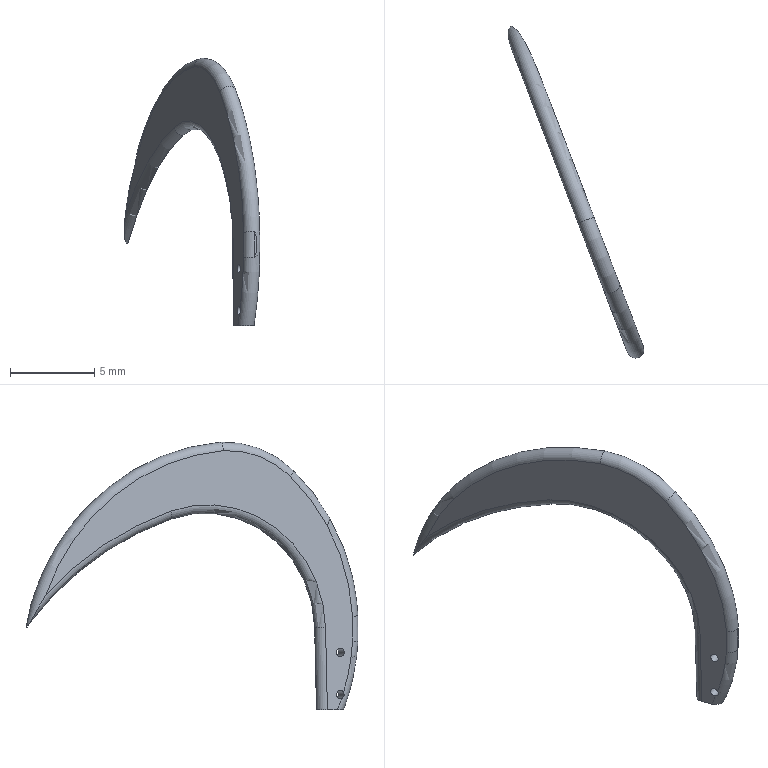Component | NX | CUTTING_BLADE | 1 solid | 16 faces | box 8.06 x 19.66 x 15.86 mm | volume 81 mm3 | torus 7 | cylinder 5 | plane 4 | commonest cylinder face diameters 1 x2 0.5 x2 12 x1
STEP:
#1=VALUE_REPRESENTATION_ITEM('',COUNT_MEASURE(0.));
#2=(LENGTH_UNIT()NAMED_UNIT(*)SI_UNIT(.MILLI.,.METRE.));
#3=UNCERTAINTY_MEASURE_WITH_UNIT(LENGTH_MEASURE(0.0508),#2,'','');
#4=(NAMED_UNIT(*)PLANE_ANGLE_UNIT()SI_UNIT($,.RADIAN.));
#5=PLANE_ANGLE_MEASURE_WITH_UNIT(PLANE_ANGLE_MEASURE(0.01745),#4);
#6=DIMENSIONAL_EXPONENTS(0.,0.,0.,0.,0.,0.,0.);
#7=(CONVERSION_BASED_UNIT('',#5)NAMED_UNIT(#6)PLANE_ANGLE_UNIT());
#8=(NAMED_UNIT(*)SI_UNIT($,.STERADIAN.)SOLID_ANGLE_UNIT());
#9=(GEOMETRIC_REPRESENTATION_CONTEXT(3)GLOBAL_UNCERTAINTY_ASSIGNED_CONTEXT((#3))GLOBAL_UNIT_ASSIGNED_CONTEXT((#2,#7,#8))REPRESENTATION_CONTEXT('',''));
#10=REPRESENTATION('',(#1),#9);
#11=VALUE_REPRESENTATION_ITEM('',COUNT_MEASURE(0.));
#12=REPRESENTATION('',(#11),#9);
#13=CARTESIAN_POINT('',(0.,0.,0.));
#14=DIRECTION('',(0.,0.,1.));
#15=DIRECTION('',(1.,0.,0.));
#16=AXIS2_PLACEMENT_3D('',#13,#14,#15);
#17=SHAPE_REPRESENTATION('',(#16),#9);
#18=CARTESIAN_POINT('',(-0.7584,2.547,-2.1));
#19=VERTEX_POINT('',#18);
#20=CARTESIAN_POINT('',(-0.8475,2.781,-2.1));
#21=DIRECTION('',(-0.9342,-0.3566,0.));
#22=DIRECTION('',(0.3566,-0.9342,0.));
#23=AXIS2_PLACEMENT_3D('',#20,#21,#22);
#24=CIRCLE('',#23,0.25);
#25=EDGE_CURVE('',#19,#19,#24,.T.);
#26=ORIENTED_EDGE('',*,*,#25,.F.);
#27=EDGE_LOOP('',(#26));
#28=FACE_BOUND('',#27,.T.);
#29=CARTESIAN_POINT('',(-1.18,3.651,-0.6366));
#30=VERTEX_POINT('',#29);
#31=CARTESIAN_POINT('',(-1.138,3.542,-5.5));
#32=VERTEX_POINT('',#31);
#33=CARTESIAN_POINT('',(-1.078,3.384,-12.534));
#34=DIRECTION('',(0.008553,-0.02241,-0.9997));
#35=VECTOR('',#34,1.);
#36=LINE('',#33,#35);
#37=EDGE_CURVE('',#30,#32,#36,.T.);
#38=ORIENTED_EDGE('',*,*,#37,.T.);
#39=CARTESIAN_POINT('',(-0.9125,2.951,-5.5));
#40=VERTEX_POINT('',#39);
#41=CARTESIAN_POINT('',(-2.44,6.953,-5.5));
#42=DIRECTION('',(0.3566,-0.9342,0.));
#43=VECTOR('',#42,1.);
#44=LINE('',#41,#43);
#45=EDGE_CURVE('',#32,#40,#44,.T.);
#46=ORIENTED_EDGE('',*,*,#45,.T.);
#47=CARTESIAN_POINT('',(-0.8194,2.707,-4.837));
#48=VERTEX_POINT('',#47);
#49=CARTESIAN_POINT('',(-4.918,13.443,-0.6896));
#50=DIRECTION('',(-0.9342,-0.3566,0.));
#51=DIRECTION('',(0.,0.,1.));
#52=AXIS2_PLACEMENT_3D('',#49,#50,#51);
#53=CIRCLE('',#52,12.217);
#54=EDGE_CURVE('',#40,#48,#53,.T.);
#55=ORIENTED_EDGE('',*,*,#54,.T.);
#56=CARTESIAN_POINT('',(-0.7734,2.587,-4.461));
#57=VERTEX_POINT('',#56);
#58=CARTESIAN_POINT('',(-0.8475,2.781,-4.6));
#59=DIRECTION('',(-0.9342,-0.3566,0.));
#60=DIRECTION('',(0.3566,-0.9342,0.));
#61=AXIS2_PLACEMENT_3D('',#58,#59,#60);
#62=CIRCLE('',#61,0.25);
#63=EDGE_CURVE('',#57,#48,#62,.T.);
#64=ORIENTED_EDGE('',*,*,#63,.F.);
#65=CARTESIAN_POINT('',(-0.5687,2.05,-1.433));
#66=VERTEX_POINT('',#65);
#67=CARTESIAN_POINT('',(-4.918,13.443,-0.6896));
#68=DIRECTION('',(-0.9342,-0.3566,0.));
#69=DIRECTION('',(0.,0.,1.));
#70=AXIS2_PLACEMENT_3D('',#67,#68,#69);
#71=CIRCLE('',#70,12.217);
#72=EDGE_CURVE('',#57,#66,#71,.T.);
#73=ORIENTED_EDGE('',*,*,#72,.T.);
#74=CARTESIAN_POINT('',(-0.5684,2.049,0.03886));
#75=VERTEX_POINT('',#74);
#76=CARTESIAN_POINT('',(-0.5687,2.05,-12.625));
#77=DIRECTION('',(0.,-0.,1.));
#78=VECTOR('',#77,1.);
#79=LINE('',#76,#78);
#80=EDGE_CURVE('',#66,#75,#79,.T.);
#81=ORIENTED_EDGE('',*,*,#80,.T.);
#82=CARTESIAN_POINT('',(-1.979,5.744,8.329));
#83=VERTEX_POINT('',#82);
#84=CARTESIAN_POINT('',(-4.918,13.443,-0.6896));
#85=DIRECTION('',(-0.9342,-0.3566,0.));
#86=DIRECTION('',(0.,0.,1.));
#87=AXIS2_PLACEMENT_3D('',#84,#85,#86);
#88=CIRCLE('',#87,12.217);
#89=EDGE_CURVE('',#75,#83,#88,.T.);
#90=ORIENTED_EDGE('',*,*,#89,.T.);
#91=CARTESIAN_POINT('',(-3.485,9.689,9.851));
#92=VERTEX_POINT('',#91);
#93=CARTESIAN_POINT('',(-3.383,9.423,4.019));
#94=DIRECTION('',(-0.9342,-0.3566,0.));
#95=DIRECTION('',(0.,0.,1.));
#96=AXIS2_PLACEMENT_3D('',#93,#94,#95);
#97=CIRCLE('',#96,5.838);
#98=EDGE_CURVE('',#83,#92,#97,.T.);
#99=ORIENTED_EDGE('',*,*,#98,.T.);
#100=CARTESIAN_POINT('',(-7.5,20.207,1.333));
#101=VERTEX_POINT('',#100);
#102=CARTESIAN_POINT('',(-3.1,8.68,-3.276));
#103=DIRECTION('',(-0.9342,-0.3566,0.));
#104=DIRECTION('',(0.,0.,1.));
#105=AXIS2_PLACEMENT_3D('',#102,#103,#104);
#106=CIRCLE('',#105,13.171);
#107=EDGE_CURVE('',#92,#101,#106,.T.);
#108=ORIENTED_EDGE('',*,*,#107,.T.);
#109=CARTESIAN_POINT('',(-4.677,12.813,6.263));
#110=VERTEX_POINT('',#109);
#111=CARTESIAN_POINT('',(-2.44,6.953,-12.625));
#112=DIRECTION('',(0.9342,0.3566,0.));
#113=DIRECTION('',(0.,0.,1.));
#114=AXIS2_PLACEMENT_3D('',#111,#112,#113);
#115=CIRCLE('',#114,19.903);
#116=EDGE_CURVE('',#101,#110,#115,.T.);
#117=ORIENTED_EDGE('',*,*,#116,.T.);
#118=CARTESIAN_POINT('',(-3.839,10.617,-0.8155));
#119=DIRECTION('',(0.9342,0.3566,0.));
#120=DIRECTION('',(0.,0.,1.));
#121=AXIS2_PLACEMENT_3D('',#118,#119,#120);
#122=CIRCLE('',#121,7.459);
#123=EDGE_CURVE('',#110,#30,#122,.T.);
#124=ORIENTED_EDGE('',*,*,#123,.T.);
#125=EDGE_LOOP('',(#38,#46,#55,#64,#73,#81,#90,#99,#108,#117,#124));
#126=FACE_BOUND('',#125,.T.);
#127=CARTESIAN_POINT('',(-2.44,6.953,-12.625));
#128=DIRECTION('',(0.9342,0.3566,0.));
#129=DIRECTION('',(0.,0.,1.));
#130=AXIS2_PLACEMENT_3D('',#127,#128,#129);
#131=PLANE('',#130);
#132=ADVANCED_FACE('',(#28,#126),#131,.F.);
#133=CARTESIAN_POINT('',(0.07677,1.761,0.06867));
#134=VERTEX_POINT('',#133);
#135=CARTESIAN_POINT('',(0.07677,1.761,-1.448));
#136=VERTEX_POINT('',#135);
#137=CARTESIAN_POINT('',(0.07677,1.761,-6.102));
#138=DIRECTION('',(-0.,0.,-1.));
#139=VECTOR('',#138,1.);
#140=LINE('',#137,#139);
#141=EDGE_CURVE('',#134,#136,#140,.T.);
#142=ORIENTED_EDGE('',*,*,#141,.T.);
#143=CARTESIAN_POINT('',(0.07677,1.761,-1.448));
#144=CARTESIAN_POINT('',(0.08034,1.763,-1.448));
#145=CARTESIAN_POINT('',(0.08395,1.764,-1.447));
#146=CARTESIAN_POINT('',(0.08729,1.765,-1.446));
#147=CARTESIAN_POINT('',(0.09154,1.767,-1.444));
#148=CARTESIAN_POINT('',(0.09549,1.769,-1.441));
#149=CARTESIAN_POINT('',(0.09903,1.77,-1.438));
#150=CARTESIAN_POINT('',(0.1054,1.772,-1.433));
#151=CARTESIAN_POINT('',(0.1108,1.774,-1.426));
#152=CARTESIAN_POINT('',(0.1155,1.776,-1.418));
#153=CARTESIAN_POINT('',(0.1308,1.782,-1.395));
#154=CARTESIAN_POINT('',(0.1405,1.786,-1.367));
#155=CARTESIAN_POINT('',(0.1489,1.789,-1.34));
#156=CARTESIAN_POINT('',(0.1867,1.803,-1.216));
#157=CARTESIAN_POINT('',(0.1985,1.808,-1.084));
#158=CARTESIAN_POINT('',(0.2072,1.811,-0.9541));
#159=CARTESIAN_POINT('',(0.2188,1.816,-0.7803));
#160=CARTESIAN_POINT('',(0.2189,1.816,-0.6051));
#161=CARTESIAN_POINT('',(0.2076,1.811,-0.4313));
#162=CARTESIAN_POINT('',(0.2019,1.809,-0.3444));
#163=CARTESIAN_POINT('',(0.1934,1.806,-0.2576));
#164=CARTESIAN_POINT('',(0.1788,1.8,-0.172));
#165=CARTESIAN_POINT('',(0.1715,1.798,-0.1292));
#166=CARTESIAN_POINT('',(0.1628,1.794,-0.08648));
#167=CARTESIAN_POINT('',(0.1505,1.79,-0.04499));
#168=CARTESIAN_POINT('',(0.146,1.788,-0.02961));
#169=CARTESIAN_POINT('',(0.1409,1.786,-0.01438));
#170=CARTESIAN_POINT('',(0.1349,1.784,0.0004269));
#171=CARTESIAN_POINT('',(0.129,1.781,0.01514));
#172=CARTESIAN_POINT('',(0.1221,1.779,0.02967));
#173=CARTESIAN_POINT('',(0.1133,1.775,0.04259));
#174=CARTESIAN_POINT('',(0.1101,1.774,0.04719));
#175=CARTESIAN_POINT('',(0.1067,1.773,0.05161));
#176=CARTESIAN_POINT('',(0.1028,1.771,0.05554));
#177=CARTESIAN_POINT('',(0.09889,1.77,0.05951));
#178=CARTESIAN_POINT('',(0.09448,1.768,0.06308));
#179=CARTESIAN_POINT('',(0.08961,1.766,0.0655));
#180=CARTESIAN_POINT('',(0.08656,1.765,0.06701));
#181=CARTESIAN_POINT('',(0.08326,1.764,0.06808));
#182=CARTESIAN_POINT('',(0.07992,1.763,0.06848));
#183=CARTESIAN_POINT('',(0.07887,1.762,0.06861));
#184=CARTESIAN_POINT('',(0.07782,1.762,0.06867));
#185=CARTESIAN_POINT('',(0.07677,1.761,0.06867));
#186=B_SPLINE_CURVE_WITH_KNOTS('',3,(#143,#144,#145,#146,#147,#148,#149,#150,#151,#152,#153,#154,#155,#156,#157,#158,#159,#160,#161,#162,#163,#164,#165,#166,#167,#168,#169,#170,#171,#172,#173,#174,#175,#176,#177,#178,#179,#180,#181,#182,#183,#184,#185),.UNSPECIFIED.,.F.,.F.,(4,3,3,3,3,3,3,3,3,3,3,3,3,3,4),(0.,0.007104,0.01617,0.03265,0.08702,0.3333,0.6626,0.8268,0.9089,0.9392,0.9695,0.9803,0.9911,0.9979,1.),.UNSPECIFIED.);
#187=EDGE_CURVE('',#136,#134,#186,.T.);
#188=ORIENTED_EDGE('',*,*,#187,.T.);
#189=EDGE_LOOP('',(#142,#188));
#190=FACE_OUTER_BOUND('',#189,.T.);
#191=CARTESIAN_POINT('',(-0.3904,1.583,-6.102));
#192=DIRECTION('',(-0.3566,0.9342,0.));
#193=DIRECTION('',(-0.,0.,-1.));
#194=AXIS2_PLACEMENT_3D('',#191,#192,#193);
#195=PLANE('',#194);
#196=ADVANCED_FACE('',(#190),#195,.F.);
#197=CARTESIAN_POINT('',(-5.429,17.586,6.197));
#198=VERTEX_POINT('',#197);
#199=CARTESIAN_POINT('',(-2.551,10.046,9.851));
#200=VERTEX_POINT('',#199);
#201=CARTESIAN_POINT('',(-2.165,9.037,-3.276));
#202=DIRECTION('',(0.9342,0.3566,0.));
#203=DIRECTION('',(0.,0.,1.));
#204=AXIS2_PLACEMENT_3D('',#201,#202,#203);
#205=CIRCLE('',#204,13.171);
#206=EDGE_CURVE('',#198,#200,#205,.T.);
#207=ORIENTED_EDGE('',*,*,#206,.T.);
#208=CARTESIAN_POINT('',(-1.044,6.1,8.329));
#209=VERTEX_POINT('',#208);
#210=CARTESIAN_POINT('',(-2.449,9.78,4.019));
#211=DIRECTION('',(0.9342,0.3566,0.));
#212=DIRECTION('',(0.,0.,1.));
#213=AXIS2_PLACEMENT_3D('',#210,#211,#212);
#214=CIRCLE('',#213,5.838);
#215=EDGE_CURVE('',#200,#209,#214,.T.);
#216=ORIENTED_EDGE('',*,*,#215,.T.);
#217=CARTESIAN_POINT('',(0.2395,2.737,2.319));
#218=VERTEX_POINT('',#217);
#219=CARTESIAN_POINT('',(-3.984,13.8,-0.6896));
#220=DIRECTION('',(0.9342,0.3566,0.));
#221=DIRECTION('',(0.,0.,1.));
#222=AXIS2_PLACEMENT_3D('',#219,#220,#221);
#223=CIRCLE('',#222,12.217);
#224=EDGE_CURVE('',#209,#218,#223,.T.);
#225=ORIENTED_EDGE('',*,*,#224,.T.);
#226=CARTESIAN_POINT('',(-3.956,13.729,8.064));
#227=VERTEX_POINT('',#226);
#228=CARTESIAN_POINT('',(-2.905,10.974,-0.8155));
#229=DIRECTION('',(-0.9342,-0.3566,0.));
#230=DIRECTION('',(0.,0.,1.));
#231=AXIS2_PLACEMENT_3D('',#228,#229,#230);
#232=CIRCLE('',#231,9.357);
#233=EDGE_CURVE('',#218,#227,#232,.T.);
#234=ORIENTED_EDGE('',*,*,#233,.T.);
#235=CARTESIAN_POINT('',(-1.506,7.309,-12.625));
#236=DIRECTION('',(-0.9342,-0.3566,0.));
#237=DIRECTION('',(0.,0.,1.));
#238=AXIS2_PLACEMENT_3D('',#235,#236,#237);
#239=CIRCLE('',#238,21.801);
#240=EDGE_CURVE('',#227,#198,#239,.T.);
#241=ORIENTED_EDGE('',*,*,#240,.T.);
#242=EDGE_LOOP('',(#207,#216,#225,#234,#241));
#243=FACE_OUTER_BOUND('',#242,.T.);
#244=CARTESIAN_POINT('',(-1.506,7.309,-12.625));
#245=DIRECTION('',(0.9342,0.3566,0.));
#246=DIRECTION('',(0.,0.,1.));
#247=AXIS2_PLACEMENT_3D('',#244,#245,#246);
#248=PLANE('',#247);
#249=ADVANCED_FACE('',(#243),#248,.T.);
#250=CARTESIAN_POINT('',(-0.8492,4.187,-5.5));
#251=VERTEX_POINT('',#250);
#252=CARTESIAN_POINT('',(-0.6709,3.72,-5.5));
#253=DIRECTION('',(0.,0.,-1.));
#254=DIRECTION('',(0.3566,-0.9342,0.));
#255=AXIS2_PLACEMENT_3D('',#252,#253,#254);
#256=ELLIPSE('',#255,0.5001,0.5);
#257=EDGE_CURVE('',#32,#251,#256,.T.);
#258=ORIENTED_EDGE('',*,*,#257,.F.);
#259=ORIENTED_EDGE('',*,*,#37,.F.);
#260=CARTESIAN_POINT('',(-0.8907,4.296,-0.6486));
#261=VERTEX_POINT('',#260);
#262=CARTESIAN_POINT('',(-0.7125,3.829,-0.6366));
#263=DIRECTION('',(-0.008553,0.02241,0.9997));
#264=DIRECTION('',(-0.3565,0.934,-0.02398));
#265=AXIS2_PLACEMENT_3D('',#262,#263,#264);
#266=CIRCLE('',#265,0.5);
#267=EDGE_CURVE('',#261,#30,#266,.T.);
#268=ORIENTED_EDGE('',*,*,#267,.F.);
#269=CARTESIAN_POINT('',(-0.8907,4.296,-0.6486));
#270=DIRECTION('',(-0.008553,0.02241,0.9997));
#271=VECTOR('',#270,1.);
#272=LINE('',#269,#271);
#273=EDGE_CURVE('',#251,#261,#272,.T.);
#274=ORIENTED_EDGE('',*,*,#273,.F.);
#275=EDGE_LOOP('',(#258,#259,#268,#274));
#276=FACE_OUTER_BOUND('',#275,.T.);
#277=CARTESIAN_POINT('',(-0.6107,3.562,-12.534));
#278=DIRECTION('',(0.008553,-0.02241,-0.9997));
#279=DIRECTION('',(0.3565,-0.934,0.02398));
#280=AXIS2_PLACEMENT_3D('',#277,#278,#279);
#281=CYLINDRICAL_SURFACE('',#280,0.5);
#282=ADVANCED_FACE('',(#276),#281,.T.);
#283=ORIENTED_EDGE('',*,*,#267,.T.);
#284=ORIENTED_EDGE('',*,*,#123,.F.);
#285=CARTESIAN_POINT('',(-4.154,12.844,5.789));
#286=VERTEX_POINT('',#285);
#287=CARTESIAN_POINT('',(-4.21,12.992,6.263));
#288=DIRECTION('',(-0.3385,0.8866,-0.3152));
#289=DIRECTION('',(0.1124,-0.2945,-0.949));
#290=AXIS2_PLACEMENT_3D('',#287,#288,#289);
#291=CIRCLE('',#290,0.5);
#292=EDGE_CURVE('',#286,#110,#291,.T.);
#293=ORIENTED_EDGE('',*,*,#292,.F.);
#294=CARTESIAN_POINT('',(-3.372,10.795,-0.8155));
#295=DIRECTION('',(-0.9342,-0.3566,0.));
#296=DIRECTION('',(0.,0.,1.));
#297=AXIS2_PLACEMENT_3D('',#294,#295,#296);
#298=CIRCLE('',#297,6.959);
#299=EDGE_CURVE('',#261,#286,#298,.T.);
#300=ORIENTED_EDGE('',*,*,#299,.F.);
#301=EDGE_LOOP('',(#283,#284,#293,#300));
#302=FACE_OUTER_BOUND('',#301,.T.);
#303=CARTESIAN_POINT('',(-3.372,10.795,-0.8155));
#304=DIRECTION('',(0.9342,0.3566,0.));
#305=DIRECTION('',(0.,0.,1.));
#306=AXIS2_PLACEMENT_3D('',#303,#304,#305);
#307=TOROIDAL_SURFACE('',#306,7.459,0.5);
#308=ADVANCED_FACE('',(#302),#307,.T.);
#309=ORIENTED_EDGE('',*,*,#116,.F.);
#310=CARTESIAN_POINT('',(-7.417,21.393,-0.6486));
#311=VERTEX_POINT('',#310);
#312=CARTESIAN_POINT('',(-7.5,20.207,1.333));
#313=CARTESIAN_POINT('',(-7.5,20.208,1.331));
#314=CARTESIAN_POINT('',(-7.501,20.209,1.329));
#315=CARTESIAN_POINT('',(-7.501,20.211,1.328));
#316=CARTESIAN_POINT('',(-7.522,20.266,1.234));
#317=CARTESIAN_POINT('',(-7.542,20.322,1.139));
#318=CARTESIAN_POINT('',(-7.559,20.377,1.044));
#319=CARTESIAN_POINT('',(-7.636,20.62,0.6261));
#320=CARTESIAN_POINT('',(-7.689,20.856,0.1886));
#321=CARTESIAN_POINT('',(-7.635,21.098,-0.2331));
#322=CARTESIAN_POINT('',(-7.622,21.158,-0.3366));
#323=CARTESIAN_POINT('',(-7.602,21.219,-0.4418));
#324=CARTESIAN_POINT('',(-7.557,21.282,-0.5333));
#325=CARTESIAN_POINT('',(-7.543,21.302,-0.5613));
#326=CARTESIAN_POINT('',(-7.526,21.322,-0.5883));
#327=CARTESIAN_POINT('',(-7.503,21.341,-0.6101));
#328=CARTESIAN_POINT('',(-7.491,21.351,-0.6221));
#329=CARTESIAN_POINT('',(-7.477,21.362,-0.6326));
#330=CARTESIAN_POINT('',(-7.461,21.372,-0.6396));
#331=CARTESIAN_POINT('',(-7.447,21.379,-0.6452));
#332=CARTESIAN_POINT('',(-7.432,21.387,-0.6486));
#333=CARTESIAN_POINT('',(-7.417,21.393,-0.6486));
#334=B_SPLINE_CURVE_WITH_KNOTS('',3,(#312,#313,#314,#315,#316,#317,#318,#319,#320,#321,#322,#323,#324,#325,#326,#327,#328,#329,#330,#331,#332,#333),.UNSPECIFIED.,.F.,.F.,(4,3,3,3,3,3,3,4),(0.,0.002895,0.1423,0.7589,0.9093,0.9549,0.9797,1.),.UNSPECIFIED.);
#335=EDGE_CURVE('',#101,#311,#334,.T.);
#336=ORIENTED_EDGE('',*,*,#335,.T.);
#337=CARTESIAN_POINT('',(-1.973,7.131,-12.625));
#338=DIRECTION('',(-0.9342,-0.3566,0.));
#339=DIRECTION('',(0.,0.,1.));
#340=AXIS2_PLACEMENT_3D('',#337,#338,#339);
#341=CIRCLE('',#340,19.403);
#342=EDGE_CURVE('',#286,#311,#341,.T.);
#343=ORIENTED_EDGE('',*,*,#342,.F.);
#344=ORIENTED_EDGE('',*,*,#292,.T.);
#345=EDGE_LOOP('',(#309,#336,#343,#344));
#346=FACE_OUTER_BOUND('',#345,.T.);
#347=CARTESIAN_POINT('',(-1.973,7.131,-12.625));
#348=DIRECTION('',(0.9342,0.3566,0.));
#349=DIRECTION('',(0.,0.,1.));
#350=AXIS2_PLACEMENT_3D('',#347,#348,#349);
#351=TOROIDAL_SURFACE('',#350,19.903,0.5);
#352=ADVANCED_FACE('',(#346),#351,.T.);
#353=ORIENTED_EDGE('',*,*,#342,.T.);
#354=CARTESIAN_POINT('',(-7.417,21.393,-0.6486));
#355=CARTESIAN_POINT('',(-7.073,21.245,0.6829));
#356=CARTESIAN_POINT('',(-6.778,20.728,1.94));
#357=CARTESIAN_POINT('',(-6.136,19.399,4.25));
#358=CARTESIAN_POINT('',(-5.8,18.558,5.29));
#359=CARTESIAN_POINT('',(-5.429,17.586,6.197));
#360=B_SPLINE_CURVE_WITH_KNOTS('',3,(#354,#355,#356,#357,#358,#359),.UNSPECIFIED.,.F.,.F.,(4,2,4),(0.,0.5,1.),.UNSPECIFIED.);
#361=EDGE_CURVE('',#311,#198,#360,.T.);
#362=ORIENTED_EDGE('',*,*,#361,.T.);
#363=ORIENTED_EDGE('',*,*,#240,.F.);
#364=CARTESIAN_POINT('',(-9.562,11.589,8.064));
#365=DIRECTION('',(0.3385,-0.8866,0.3152));
#366=DIRECTION('',(-0.1124,0.2945,0.949));
#367=AXIS2_PLACEMENT_3D('',#364,#365,#366);
#368=CIRCLE('',#367,6.);
#369=EDGE_CURVE('',#286,#227,#368,.T.);
#370=ORIENTED_EDGE('',*,*,#369,.F.);
#371=EDGE_LOOP('',(#353,#362,#363,#370));
#372=FACE_OUTER_BOUND('',#371,.T.);
#373=CARTESIAN_POINT('',(-7.111,5.17,-12.625));
#374=DIRECTION('',(0.9342,0.3566,0.));
#375=DIRECTION('',(0.,0.,1.));
#376=AXIS2_PLACEMENT_3D('',#373,#374,#375);
#377=TOROIDAL_SURFACE('',#376,21.801,6.);
#378=ADVANCED_FACE('',(#372),#377,.T.);
#379=ORIENTED_EDGE('',*,*,#233,.F.);
#380=CARTESIAN_POINT('',(0.3852,2.352,-0.5941));
#381=VERTEX_POINT('',#380);
#382=CARTESIAN_POINT('',(0.2395,2.737,2.319));
#383=CARTESIAN_POINT('',(0.331,2.498,1.365));
#384=CARTESIAN_POINT('',(0.3815,2.362,0.3811));
#385=CARTESIAN_POINT('',(0.3852,2.352,-0.5941));
#386=B_SPLINE_CURVE_WITH_KNOTS('',3,(#382,#383,#384,#385),.UNSPECIFIED.,.F.,.F.,(4,4),(0.,1.),.UNSPECIFIED.);
#387=EDGE_CURVE('',#218,#381,#386,.T.);
#388=ORIENTED_EDGE('',*,*,#387,.T.);
#389=CARTESIAN_POINT('',(-5.174,0.09486,-0.5911));
#390=DIRECTION('',(0.008553,-0.02241,-0.9997));
#391=DIRECTION('',(0.3565,-0.934,0.02398));
#392=AXIS2_PLACEMENT_3D('',#389,#390,#391);
#393=CIRCLE('',#392,6.);
#394=EDGE_CURVE('',#261,#381,#393,.T.);
#395=ORIENTED_EDGE('',*,*,#394,.F.);
#396=ORIENTED_EDGE('',*,*,#299,.T.);
#397=ORIENTED_EDGE('',*,*,#369,.T.);
#398=EDGE_LOOP('',(#379,#388,#395,#396,#397));
#399=FACE_OUTER_BOUND('',#398,.T.);
#400=CARTESIAN_POINT('',(-8.51,8.834,-0.8155));
#401=DIRECTION('',(0.9342,0.3566,0.));
#402=DIRECTION('',(0.,0.,1.));
#403=AXIS2_PLACEMENT_3D('',#400,#401,#402);
#404=TOROIDAL_SURFACE('',#403,9.357,6.);
#405=ADVANCED_FACE('',(#399),#404,.T.);
#406=CARTESIAN_POINT('',(0.05222,3.005,-5.5));
#407=VERTEX_POINT('',#406);
#408=CARTESIAN_POINT('',(-5.132,-0.01516,-5.5));
#409=DIRECTION('',(0.,0.,-1.));
#410=DIRECTION('',(0.3566,-0.9342,0.));
#411=AXIS2_PLACEMENT_3D('',#408,#409,#410);
#412=ELLIPSE('',#411,6.002,6.);
#413=EDGE_CURVE('',#251,#407,#412,.T.);
#414=ORIENTED_EDGE('',*,*,#413,.F.);
#415=ORIENTED_EDGE('',*,*,#273,.T.);
#416=ORIENTED_EDGE('',*,*,#394,.T.);
#417=CARTESIAN_POINT('',(0.3852,2.352,-0.5941));
#418=CARTESIAN_POINT('',(0.3916,2.334,-2.262));
#419=CARTESIAN_POINT('',(0.3184,2.561,-3.913));
#420=CARTESIAN_POINT('',(0.05222,3.005,-5.5));
#421=B_SPLINE_CURVE_WITH_KNOTS('',3,(#417,#418,#419,#420),.UNSPECIFIED.,.F.,.F.,(4,4),(0.,1.),.UNSPECIFIED.);
#422=EDGE_CURVE('',#381,#407,#421,.T.);
#423=ORIENTED_EDGE('',*,*,#422,.T.);
#424=EDGE_LOOP('',(#414,#415,#416,#423));
#425=FACE_BOUND('',#424,.T.);
#426=CARTESIAN_POINT('',(-0.002817,3.103,-4.85));
#427=VERTEX_POINT('',#426);
#428=CARTESIAN_POINT('',(-0.002817,3.103,-4.85));
#429=CARTESIAN_POINT('',(-0.01776,3.128,-4.85));
#430=CARTESIAN_POINT('',(-0.03308,3.153,-4.845));
#431=CARTESIAN_POINT('',(-0.04748,3.176,-4.835));
#432=CARTESIAN_POINT('',(-0.06187,3.199,-4.826));
#433=CARTESIAN_POINT('',(-0.07575,3.221,-4.812));
#434=CARTESIAN_POINT('',(-0.08784,3.24,-4.793));
#435=CARTESIAN_POINT('',(-0.09988,3.259,-4.775));
#436=CARTESIAN_POINT('',(-0.1105,3.276,-4.753));
#437=CARTESIAN_POINT('',(-0.1186,3.288,-4.729));
#438=CARTESIAN_POINT('',(-0.1266,3.301,-4.705));
#439=CARTESIAN_POINT('',(-0.1324,3.31,-4.678));
#440=CARTESIAN_POINT('',(-0.1355,3.315,-4.65));
#441=CARTESIAN_POINT('',(-0.1385,3.32,-4.623));
#442=CARTESIAN_POINT('',(-0.1389,3.32,-4.595));
#443=CARTESIAN_POINT('',(-0.1367,3.317,-4.567));
#444=CARTESIAN_POINT('',(-0.1346,3.314,-4.54));
#445=CARTESIAN_POINT('',(-0.1298,3.307,-4.514));
#446=CARTESIAN_POINT('',(-0.1229,3.297,-4.489));
#447=CARTESIAN_POINT('',(-0.116,3.287,-4.465));
#448=CARTESIAN_POINT('',(-0.1067,3.273,-4.442));
#449=CARTESIAN_POINT('',(-0.09596,3.256,-4.423));
#450=CARTESIAN_POINT('',(-0.08497,3.239,-4.403));
#451=CARTESIAN_POINT('',(-0.07214,3.219,-4.387));
#452=CARTESIAN_POINT('',(-0.05859,3.198,-4.375));
#453=CARTESIAN_POINT('',(-0.04477,3.176,-4.362));
#454=CARTESIAN_POINT('',(-0.02982,3.152,-4.355));
#455=CARTESIAN_POINT('',(-0.01501,3.127,-4.351));
#456=CARTESIAN_POINT('',(-0.00006101,3.103,-4.348));
#457=CARTESIAN_POINT('',(0.01517,3.077,-4.35));
#458=CARTESIAN_POINT('',(0.02941,3.053,-4.357));
#459=CARTESIAN_POINT('',(0.0436,3.029,-4.364));
#460=CARTESIAN_POINT('',(0.05721,3.005,-4.375));
#461=CARTESIAN_POINT('',(0.06915,2.984,-4.391));
#462=CARTESIAN_POINT('',(0.08095,2.964,-4.406));
#463=CARTESIAN_POINT('',(0.09144,2.945,-4.426));
#464=CARTESIAN_POINT('',(0.09982,2.93,-4.449));
#465=CARTESIAN_POINT('',(0.1081,2.915,-4.471));
#466=CARTESIAN_POINT('',(0.1145,2.903,-4.496));
#467=CARTESIAN_POINT('',(0.1186,2.895,-4.523));
#468=CARTESIAN_POINT('',(0.1227,2.887,-4.55));
#469=CARTESIAN_POINT('',(0.1246,2.884,-4.578));
#470=CARTESIAN_POINT('',(0.1242,2.884,-4.606));
#471=CARTESIAN_POINT('',(0.1238,2.885,-4.633));
#472=CARTESIAN_POINT('',(0.1212,2.889,-4.661));
#473=CARTESIAN_POINT('',(0.1164,2.898,-4.687));
#474=CARTESIAN_POINT('',(0.1116,2.907,-4.713));
#475=CARTESIAN_POINT('',(0.1045,2.919,-4.738));
#476=CARTESIAN_POINT('',(0.09575,2.935,-4.759));
#477=CARTESIAN_POINT('',(0.08694,2.95,-4.781));
#478=CARTESIAN_POINT('',(0.07615,2.969,-4.799));
#479=CARTESIAN_POINT('',(0.06419,2.99,-4.814));
#480=CARTESIAN_POINT('',(0.05212,3.011,-4.828));
#481=CARTESIAN_POINT('',(0.03852,3.034,-4.839));
#482=CARTESIAN_POINT('',(0.02446,3.058,-4.844));
#483=CARTESIAN_POINT('',(0.01558,3.073,-4.848));
#484=CARTESIAN_POINT('',(0.006387,3.088,-4.85));
#485=CARTESIAN_POINT('',(-0.002817,3.103,-4.85));
#486=B_SPLINE_CURVE_WITH_KNOTS('',3,(#428,#429,#430,#431,#432,#433,#434,#435,#436,#437,#438,#439,#440,#441,#442,#443,#444,#445,#446,#447,#448,#449,#450,#451,#452,#453,#454,#455,#456,#457,#458,#459,#460,#461,#462,#463,#464,#465,#466,#467,#468,#469,#470,#471,#472,#473,#474,#475,#476,#477,#478,#479,#480,#481,#482,#483,#484,#485),.UNSPECIFIED.,.T.,.F.,(1,3,3,3,3,3,3,3,3,3,3,3,3,3,3,3,3,3,3,3,3,1),(-0.03358,0.,0.05502,0.1101,0.1648,0.2186,0.2711,0.3231,0.3755,0.429,0.4836,0.5386,0.5935,0.6476,0.7011,0.7542,0.8069,0.8598,0.9128,0.9664,1.,1.055),.UNSPECIFIED.);
#487=EDGE_CURVE('',#427,#427,#486,.T.);
#488=ORIENTED_EDGE('',*,*,#487,.F.);
#489=EDGE_LOOP('',(#488));
#490=FACE_BOUND('',#489,.T.);
#491=CARTESIAN_POINT('',(0.007024,3.107,-2.35));
#492=VERTEX_POINT('',#491);
#493=CARTESIAN_POINT('',(0.007024,3.107,-2.35));
#494=CARTESIAN_POINT('',(-0.007619,3.132,-2.35));
#495=CARTESIAN_POINT('',(-0.02263,3.157,-2.345));
#496=CARTESIAN_POINT('',(-0.03675,3.18,-2.336));
#497=CARTESIAN_POINT('',(-0.05086,3.203,-2.326));
#498=CARTESIAN_POINT('',(-0.06447,3.225,-2.312));
#499=CARTESIAN_POINT('',(-0.07633,3.244,-2.294));
#500=CARTESIAN_POINT('',(-0.08815,3.263,-2.276));
#501=CARTESIAN_POINT('',(-0.09856,3.28,-2.254));
#502=CARTESIAN_POINT('',(-0.1066,3.293,-2.229));
#503=CARTESIAN_POINT('',(-0.1144,3.305,-2.205));
#504=CARTESIAN_POINT('',(-0.1202,3.314,-2.178));
#505=CARTESIAN_POINT('',(-0.1232,3.319,-2.151));
#506=CARTESIAN_POINT('',(-0.1262,3.324,-2.124));
#507=CARTESIAN_POINT('',(-0.1266,3.325,-2.095));
#508=CARTESIAN_POINT('',(-0.1245,3.322,-2.068));
#509=CARTESIAN_POINT('',(-0.1224,3.319,-2.041));
#510=CARTESIAN_POINT('',(-0.1178,3.312,-2.014));
#511=CARTESIAN_POINT('',(-0.111,3.302,-1.989));
#512=CARTESIAN_POINT('',(-0.1042,3.291,-1.965));
#513=CARTESIAN_POINT('',(-0.09508,3.277,-1.942));
#514=CARTESIAN_POINT('',(-0.08448,3.261,-1.923));
#515=CARTESIAN_POINT('',(-0.07368,3.244,-1.903));
#516=CARTESIAN_POINT('',(-0.06107,3.224,-1.887));
#517=CARTESIAN_POINT('',(-0.04775,3.202,-1.875));
#518=CARTESIAN_POINT('',(-0.03419,3.18,-1.862));
#519=CARTESIAN_POINT('',(-0.01953,3.156,-1.854));
#520=CARTESIAN_POINT('',(-0.004992,3.131,-1.851));
#521=CARTESIAN_POINT('',(0.009653,3.107,-1.848));
#522=CARTESIAN_POINT('',(0.02457,3.081,-1.85));
#523=CARTESIAN_POINT('',(0.03852,3.057,-1.857));
#524=CARTESIAN_POINT('',(0.05242,3.032,-1.863));
#525=CARTESIAN_POINT('',(0.06575,3.009,-1.875));
#526=CARTESIAN_POINT('',(0.07744,2.988,-1.891));
#527=CARTESIAN_POINT('',(0.08901,2.967,-1.906));
#528=CARTESIAN_POINT('',(0.0993,2.948,-1.926));
#529=CARTESIAN_POINT('',(0.1075,2.933,-1.948));
#530=CARTESIAN_POINT('',(0.1156,2.918,-1.97));
#531=CARTESIAN_POINT('',(0.122,2.906,-1.996));
#532=CARTESIAN_POINT('',(0.126,2.898,-2.023));
#533=CARTESIAN_POINT('',(0.1301,2.89,-2.049));
#534=CARTESIAN_POINT('',(0.132,2.886,-2.077));
#535=CARTESIAN_POINT('',(0.1316,2.887,-2.105));
#536=CARTESIAN_POINT('',(0.1312,2.887,-2.133));
#537=CARTESIAN_POINT('',(0.1286,2.892,-2.161));
#538=CARTESIAN_POINT('',(0.1239,2.901,-2.187));
#539=CARTESIAN_POINT('',(0.1192,2.909,-2.213));
#540=CARTESIAN_POINT('',(0.1123,2.922,-2.238));
#541=CARTESIAN_POINT('',(0.1037,2.938,-2.259));
#542=CARTESIAN_POINT('',(0.09511,2.953,-2.281));
#543=CARTESIAN_POINT('',(0.08452,2.972,-2.299));
#544=CARTESIAN_POINT('',(0.07278,2.993,-2.314));
#545=CARTESIAN_POINT('',(0.06094,3.014,-2.328));
#546=CARTESIAN_POINT('',(0.0476,3.037,-2.339));
#547=CARTESIAN_POINT('',(0.03379,3.061,-2.344));
#548=CARTESIAN_POINT('',(0.02508,3.076,-2.348));
#549=CARTESIAN_POINT('',(0.01606,3.092,-2.35));
#550=CARTESIAN_POINT('',(0.007024,3.107,-2.35));
#551=B_SPLINE_CURVE_WITH_KNOTS('',3,(#493,#494,#495,#496,#497,#498,#499,#500,#501,#502,#503,#504,#505,#506,#507,#508,#509,#510,#511,#512,#513,#514,#515,#516,#517,#518,#519,#520,#521,#522,#523,#524,#525,#526,#527,#528,#529,#530,#531,#532,#533,#534,#535,#536,#537,#538,#539,#540,#541,#542,#543,#544,#545,#546,#547,#548,#549,#550),.UNSPECIFIED.,.T.,.F.,(1,3,3,3,3,3,3,3,3,3,3,3,3,3,3,3,3,3,3,3,3,1),(-0.03355,0.,0.05488,0.1098,0.1644,0.2182,0.2709,0.323,0.3756,0.4291,0.4836,0.5385,0.5932,0.6473,0.7008,0.7539,0.8068,0.8597,0.9129,0.9664,1.,1.055),.UNSPECIFIED.);
#552=EDGE_CURVE('',#492,#492,#551,.T.);
#553=ORIENTED_EDGE('',*,*,#552,.F.);
#554=EDGE_LOOP('',(#553));
#555=FACE_BOUND('',#554,.T.);
#556=CARTESIAN_POINT('',(-5.174,0.09486,-0.5911));
#557=DIRECTION('',(0.008553,-0.02241,-0.9997));
#558=DIRECTION('',(0.3565,-0.934,0.02398));
#559=AXIS2_PLACEMENT_3D('',#556,#557,#558);
#560=CYLINDRICAL_SURFACE('',#559,6.);
#561=ADVANCED_FACE('',(#425,#490,#555),#560,.T.);
#562=ORIENTED_EDGE('',*,*,#80,.F.);
#563=CARTESIAN_POINT('',(-0.5687,2.05,-1.433));
#564=CARTESIAN_POINT('',(-0.5665,2.045,-1.433));
#565=CARTESIAN_POINT('',(-0.5643,2.039,-1.433));
#566=CARTESIAN_POINT('',(-0.5619,2.033,-1.433));
#567=CARTESIAN_POINT('',(-0.5401,1.982,-1.435));
#568=CARTESIAN_POINT('',(-0.509,1.933,-1.437));
#569=CARTESIAN_POINT('',(-0.4713,1.892,-1.438));
#570=CARTESIAN_POINT('',(-0.4336,1.851,-1.44));
#571=CARTESIAN_POINT('',(-0.3883,1.815,-1.441));
#572=CARTESIAN_POINT('',(-0.339,1.789,-1.443));
#573=CARTESIAN_POINT('',(-0.2897,1.762,-1.444));
#574=CARTESIAN_POINT('',(-0.2352,1.744,-1.445));
#575=CARTESIAN_POINT('',(-0.1799,1.735,-1.446));
#576=CARTESIAN_POINT('',(-0.1246,1.726,-1.447));
#577=CARTESIAN_POINT('',(-0.06709,1.727,-1.447));
#578=CARTESIAN_POINT('',(-0.01203,1.737,-1.448));
#579=CARTESIAN_POINT('',(0.01821,1.742,-1.448));
#580=CARTESIAN_POINT('',(0.04806,1.75,-1.448));
#581=CARTESIAN_POINT('',(0.07677,1.761,-1.448));
#582=B_SPLINE_CURVE_WITH_KNOTS('',3,(#563,#564,#565,#566,#567,#568,#569,#570,#571,#572,#573,#574,#575,#576,#577,#578,#579,#580,#581),.UNSPECIFIED.,.F.,.F.,(4,3,3,3,3,3,4),(0.,0.02319,0.238,0.4529,0.6677,0.8824,1.),.UNSPECIFIED.);
#583=EDGE_CURVE('',#66,#136,#582,.T.);
#584=ORIENTED_EDGE('',*,*,#583,.T.);
#585=ORIENTED_EDGE('',*,*,#141,.F.);
#586=CARTESIAN_POINT('',(-0.5684,2.049,0.03886));
#587=CARTESIAN_POINT('',(-0.4752,1.805,0.05447));
#588=CARTESIAN_POINT('',(-0.1678,1.668,0.06867));
#589=CARTESIAN_POINT('',(0.07677,1.761,0.06867));
#590=B_SPLINE_CURVE_WITH_KNOTS('',3,(#586,#587,#588,#589),.UNSPECIFIED.,.F.,.F.,(4,4),(0.,1.),.UNSPECIFIED.);
#591=EDGE_CURVE('',#75,#134,#590,.T.);
#592=ORIENTED_EDGE('',*,*,#591,.F.);
#593=EDGE_LOOP('',(#562,#584,#585,#592));
#594=FACE_OUTER_BOUND('',#593,.T.);
#595=CARTESIAN_POINT('',(-0.1015,2.229,-12.625));
#596=DIRECTION('',(0.,-0.,1.));
#597=DIRECTION('',(-0.3566,0.9342,0.));
#598=AXIS2_PLACEMENT_3D('',#595,#596,#597);
#599=CYLINDRICAL_SURFACE('',#598,0.5);
#600=ADVANCED_FACE('',(#594),#599,.T.);
#601=CARTESIAN_POINT('',(0.05222,3.005,-5.5));
#602=CARTESIAN_POINT('',(0.04205,2.946,-5.5));
#603=CARTESIAN_POINT('',(0.02175,2.888,-5.5));
#604=CARTESIAN_POINT('',(-0.007697,2.836,-5.5));
#605=CARTESIAN_POINT('',(-0.0368,2.784,-5.5));
#606=CARTESIAN_POINT('',(-0.07582,2.737,-5.5));
#607=CARTESIAN_POINT('',(-0.1215,2.699,-5.5));
#608=CARTESIAN_POINT('',(-0.1636,2.664,-5.5));
#609=CARTESIAN_POINT('',(-0.2127,2.637,-5.5));
#610=CARTESIAN_POINT('',(-0.2643,2.619,-5.5));
#611=CARTESIAN_POINT('',(-0.3135,2.601,-5.5));
#612=CARTESIAN_POINT('',(-0.3664,2.592,-5.5));
#613=CARTESIAN_POINT('',(-0.4185,2.592,-5.5));
#614=CARTESIAN_POINT('',(-0.4708,2.592,-5.5));
#615=CARTESIAN_POINT('',(-0.5237,2.601,-5.5));
#616=CARTESIAN_POINT('',(-0.5732,2.618,-5.5));
#617=CARTESIAN_POINT('',(-0.625,2.635,-5.5));
#618=CARTESIAN_POINT('',(-0.6746,2.661,-5.5));
#619=CARTESIAN_POINT('',(-0.7185,2.694,-5.5));
#620=CARTESIAN_POINT('',(-0.7656,2.728,-5.5));
#621=CARTESIAN_POINT('',(-0.8075,2.771,-5.5));
#622=CARTESIAN_POINT('',(-0.8415,2.819,-5.5));
#623=CARTESIAN_POINT('',(-0.8707,2.859,-5.5));
#624=CARTESIAN_POINT('',(-0.8947,2.904,-5.5));
#625=CARTESIAN_POINT('',(-0.9125,2.951,-5.5));
#626=B_SPLINE_CURVE_WITH_KNOTS('',3,(#601,#602,#603,#604,#605,#606,#607,#608,#609,#610,#611,#612,#613,#614,#615,#616,#617,#618,#619,#620,#621,#622,#623,#624,#625),.UNSPECIFIED.,.F.,.F.,(4,3,3,3,3,3,3,3,4),(0.,0.1361,0.2706,0.3945,0.5126,0.6308,0.7543,0.8867,1.),.UNSPECIFIED.);
#627=EDGE_CURVE('',#407,#40,#626,.T.);
#628=ORIENTED_EDGE('',*,*,#627,.F.);
#629=ORIENTED_EDGE('',*,*,#422,.F.);
#630=ORIENTED_EDGE('',*,*,#387,.F.);
#631=ORIENTED_EDGE('',*,*,#224,.F.);
#632=CARTESIAN_POINT('',(-1.511,5.922,8.329));
#633=DIRECTION('',(-0.2633,0.6897,0.6746));
#634=DIRECTION('',(-0.2406,0.6302,-0.7382));
#635=AXIS2_PLACEMENT_3D('',#632,#633,#634);
#636=CIRCLE('',#635,0.5);
#637=EDGE_CURVE('',#83,#209,#636,.T.);
#638=ORIENTED_EDGE('',*,*,#637,.F.);
#639=ORIENTED_EDGE('',*,*,#89,.F.);
#640=ORIENTED_EDGE('',*,*,#591,.T.);
#641=ORIENTED_EDGE('',*,*,#187,.F.);
#642=ORIENTED_EDGE('',*,*,#583,.F.);
#643=ORIENTED_EDGE('',*,*,#72,.F.);
#644=CARTESIAN_POINT('',(-0.8194,2.707,-4.837));
#645=CARTESIAN_POINT('',(-0.8162,2.699,-4.834));
#646=CARTESIAN_POINT('',(-0.813,2.691,-4.831));
#647=CARTESIAN_POINT('',(-0.8097,2.683,-4.827));
#648=CARTESIAN_POINT('',(-0.8004,2.661,-4.816));
#649=CARTESIAN_POINT('',(-0.7908,2.64,-4.801));
#650=CARTESIAN_POINT('',(-0.7823,2.623,-4.783));
#651=CARTESIAN_POINT('',(-0.7734,2.605,-4.764));
#652=CARTESIAN_POINT('',(-0.7656,2.589,-4.741));
#653=CARTESIAN_POINT('',(-0.7603,2.577,-4.716));
#654=CARTESIAN_POINT('',(-0.7549,2.565,-4.692));
#655=CARTESIAN_POINT('',(-0.7518,2.557,-4.664));
#656=CARTESIAN_POINT('',(-0.7512,2.553,-4.637));
#657=CARTESIAN_POINT('',(-0.7507,2.549,-4.609));
#658=CARTESIAN_POINT('',(-0.7525,2.549,-4.581));
#659=CARTESIAN_POINT('',(-0.7559,2.553,-4.554));
#660=CARTESIAN_POINT('',(-0.7594,2.557,-4.527));
#661=CARTESIAN_POINT('',(-0.7646,2.565,-4.5));
#662=CARTESIAN_POINT('',(-0.77,2.578,-4.476));
#663=CARTESIAN_POINT('',(-0.7711,2.581,-4.471));
#664=CARTESIAN_POINT('',(-0.7723,2.584,-4.466));
#665=CARTESIAN_POINT('',(-0.7734,2.587,-4.461));
#666=B_SPLINE_CURVE_WITH_KNOTS('',3,(#644,#645,#646,#647,#648,#649,#650,#651,#652,#653,#654,#655,#656,#657,#658,#659,#660,#661,#662,#663,#664,#665),.UNSPECIFIED.,.F.,.F.,(4,3,3,3,3,3,3,4),(0.,0.06035,0.2338,0.4165,0.5995,0.7797,0.9628,1.),.UNSPECIFIED.);
#667=EDGE_CURVE('',#48,#57,#666,.T.);
#668=ORIENTED_EDGE('',*,*,#667,.F.);
#669=ORIENTED_EDGE('',*,*,#54,.F.);
#670=EDGE_LOOP('',(#628,#629,#630,#631,#638,#639,#640,#641,#642,#643,#668,#669));
#671=FACE_OUTER_BOUND('',#670,.T.);
#672=CARTESIAN_POINT('',(-4.451,13.622,-0.6896));
#673=DIRECTION('',(0.9342,0.3566,0.));
#674=DIRECTION('',(0.,0.,1.));
#675=AXIS2_PLACEMENT_3D('',#672,#673,#674);
#676=TOROIDAL_SURFACE('',#675,12.217,0.5);
#677=ADVANCED_FACE('',(#671),#676,.T.);
#678=ORIENTED_EDGE('',*,*,#335,.F.);
#679=ORIENTED_EDGE('',*,*,#107,.F.);
#680=CARTESIAN_POINT('',(-3.026,9.891,10.35));
#681=VERTEX_POINT('',#680);
#682=CARTESIAN_POINT('',(-3.026,9.891,10.35));
#683=CARTESIAN_POINT('',(-3.271,9.797,10.35));
#684=CARTESIAN_POINT('',(-3.489,9.701,10.112));
#685=CARTESIAN_POINT('',(-3.485,9.689,9.851));
#686=B_SPLINE_CURVE_WITH_KNOTS('',3,(#682,#683,#684,#685),.UNSPECIFIED.,.F.,.F.,(4,4),(0.,1.),.UNSPECIFIED.);
#687=EDGE_CURVE('',#681,#92,#686,.T.);
#688=ORIENTED_EDGE('',*,*,#687,.F.);
#689=CARTESIAN_POINT('',(-2.551,10.046,9.851));
#690=CARTESIAN_POINT('',(-2.555,10.058,10.112));
#691=CARTESIAN_POINT('',(-2.782,9.984,10.35));
#692=CARTESIAN_POINT('',(-3.026,9.891,10.35));
#693=B_SPLINE_CURVE_WITH_KNOTS('',3,(#689,#690,#691,#692),.UNSPECIFIED.,.F.,.F.,(4,4),(0.,1.),.UNSPECIFIED.);
#694=EDGE_CURVE('',#200,#681,#693,.T.);
#695=ORIENTED_EDGE('',*,*,#694,.F.);
#696=ORIENTED_EDGE('',*,*,#206,.F.);
#697=ORIENTED_EDGE('',*,*,#361,.F.);
#698=EDGE_LOOP('',(#678,#679,#688,#695,#696,#697));
#699=FACE_OUTER_BOUND('',#698,.T.);
#700=CARTESIAN_POINT('',(-2.633,8.859,-3.276));
#701=DIRECTION('',(0.9342,0.3566,0.));
#702=DIRECTION('',(0.,0.,1.));
#703=AXIS2_PLACEMENT_3D('',#700,#701,#702);
#704=TOROIDAL_SURFACE('',#703,13.171,0.5);
#705=ADVANCED_FACE('',(#699),#704,.T.);
#706=ORIENTED_EDGE('',*,*,#637,.T.);
#707=ORIENTED_EDGE('',*,*,#215,.F.);
#708=ORIENTED_EDGE('',*,*,#694,.T.);
#709=ORIENTED_EDGE('',*,*,#687,.T.);
#710=ORIENTED_EDGE('',*,*,#98,.F.);
#711=EDGE_LOOP('',(#706,#707,#708,#709,#710));
#712=FACE_OUTER_BOUND('',#711,.T.);
#713=CARTESIAN_POINT('',(-2.916,9.601,4.019));
#714=DIRECTION('',(0.9342,0.3566,0.));
#715=DIRECTION('',(0.,0.,1.));
#716=AXIS2_PLACEMENT_3D('',#713,#714,#715);
#717=TOROIDAL_SURFACE('',#716,5.838,0.5);
#718=ADVANCED_FACE('',(#712),#717,.T.);
#719=ORIENTED_EDGE('',*,*,#552,.T.);
#720=EDGE_LOOP('',(#719));
#721=FACE_BOUND('',#720,.T.);
#722=ORIENTED_EDGE('',*,*,#25,.T.);
#723=EDGE_LOOP('',(#722));
#724=FACE_BOUND('',#723,.T.);
#725=CARTESIAN_POINT('',(0.8025,3.411,-2.1));
#726=DIRECTION('',(-0.9342,-0.3566,0.));
#727=DIRECTION('',(0.,0.,-1.));
#728=AXIS2_PLACEMENT_3D('',#725,#726,#727);
#729=CYLINDRICAL_SURFACE('',#728,0.25);
#730=ADVANCED_FACE('',(#721,#724),#729,.F.);
#731=ORIENTED_EDGE('',*,*,#487,.T.);
#732=EDGE_LOOP('',(#731));
#733=FACE_BOUND('',#732,.T.);
#734=ORIENTED_EDGE('',*,*,#667,.T.);
#735=ORIENTED_EDGE('',*,*,#63,.T.);
#736=EDGE_LOOP('',(#734,#735));
#737=FACE_BOUND('',#736,.T.);
#738=CARTESIAN_POINT('',(0.8025,3.411,-4.6));
#739=DIRECTION('',(-0.9342,-0.3566,0.));
#740=DIRECTION('',(0.,0.,-1.));
#741=AXIS2_PLACEMENT_3D('',#738,#739,#740);
#742=CYLINDRICAL_SURFACE('',#741,0.25);
#743=ADVANCED_FACE('',(#733,#737),#742,.F.);
#744=ORIENTED_EDGE('',*,*,#257,.T.);
#745=ORIENTED_EDGE('',*,*,#413,.T.);
#746=ORIENTED_EDGE('',*,*,#627,.T.);
#747=ORIENTED_EDGE('',*,*,#45,.F.);
#748=EDGE_LOOP('',(#744,#745,#746,#747));
#749=FACE_OUTER_BOUND('',#748,.T.);
#750=CARTESIAN_POINT('',(-0.2845,2.708,-5.5));
#751=DIRECTION('',(0.,0.,1.));
#752=DIRECTION('',(-0.9342,-0.3566,0.));
#753=AXIS2_PLACEMENT_3D('',#750,#751,#752);
#754=PLANE('',#753);
#755=ADVANCED_FACE('',(#749),#754,.F.);
#756=CLOSED_SHELL('',(#132,#196,#249,#282,#308,#352,#378,#405,#561,#600,#677,#705,#718,#730,#743,#755));
#757=MANIFOLD_SOLID_BREP('',#756);
#758=ADVANCED_BREP_SHAPE_REPRESENTATION('',(#757),#9);
#759=SHAPE_REPRESENTATION_RELATIONSHIP('','',#17,#758);
#760=PRESENTATION_LAYER_ASSIGNMENT('','',(#757));
#761=COLOUR_RGB('',0.5961,0.6667,0.6863);
#762=FILL_AREA_STYLE_COLOUR('',#761);
#763=FILL_AREA_STYLE('',(#762));
#764=SURFACE_STYLE_FILL_AREA(#763);
#765=SURFACE_SIDE_STYLE('',(#764));
#766=SURFACE_STYLE_USAGE(.BOTH.,#765);
#767=PRESENTATION_STYLE_ASSIGNMENT((#766));
#768=STYLED_ITEM('',(#767),#757);
#769=COLOUR_RGB('',1.,0.8627,0.2275);
#770=FILL_AREA_STYLE_COLOUR('',#769);
#771=FILL_AREA_STYLE('',(#770));
#772=SURFACE_STYLE_FILL_AREA(#771);
#773=SURFACE_SIDE_STYLE('',(#772));
#774=SURFACE_STYLE_USAGE(.BOTH.,#773);
#775=PRESENTATION_STYLE_ASSIGNMENT((#774));
#776=OVER_RIDING_STYLED_ITEM('',(#775),#132,#768);
#777=FILL_AREA_STYLE_COLOUR('',#769);
#778=FILL_AREA_STYLE('',(#777));
#779=SURFACE_STYLE_FILL_AREA(#778);
#780=SURFACE_SIDE_STYLE('',(#779));
#781=SURFACE_STYLE_USAGE(.BOTH.,#780);
#782=PRESENTATION_STYLE_ASSIGNMENT((#781));
#783=OVER_RIDING_STYLED_ITEM('',(#782),#196,#768);
#784=FILL_AREA_STYLE_COLOUR('',#769);
#785=FILL_AREA_STYLE('',(#784));
#786=SURFACE_STYLE_FILL_AREA(#785);
#787=SURFACE_SIDE_STYLE('',(#786));
#788=SURFACE_STYLE_USAGE(.BOTH.,#787);
#789=PRESENTATION_STYLE_ASSIGNMENT((#788));
#790=OVER_RIDING_STYLED_ITEM('',(#789),#249,#768);
#791=MECHANICAL_DESIGN_GEOMETRIC_PRESENTATION_REPRESENTATION('',(#768,#776,#783,#790),#9);